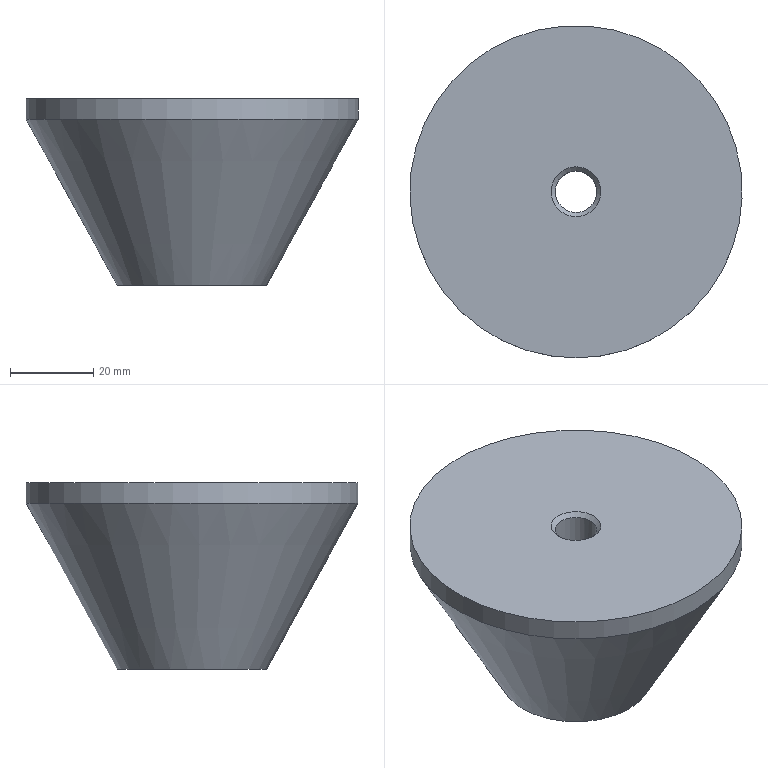Component | NX | CH3404_10-1 | 1 solid | 9 faces | volume 129483 mm3 | cylinder 4 | plane 3 | cone 2 | commonest cylinder face diameters 10 x1 80 x1 30 x1 4 x1